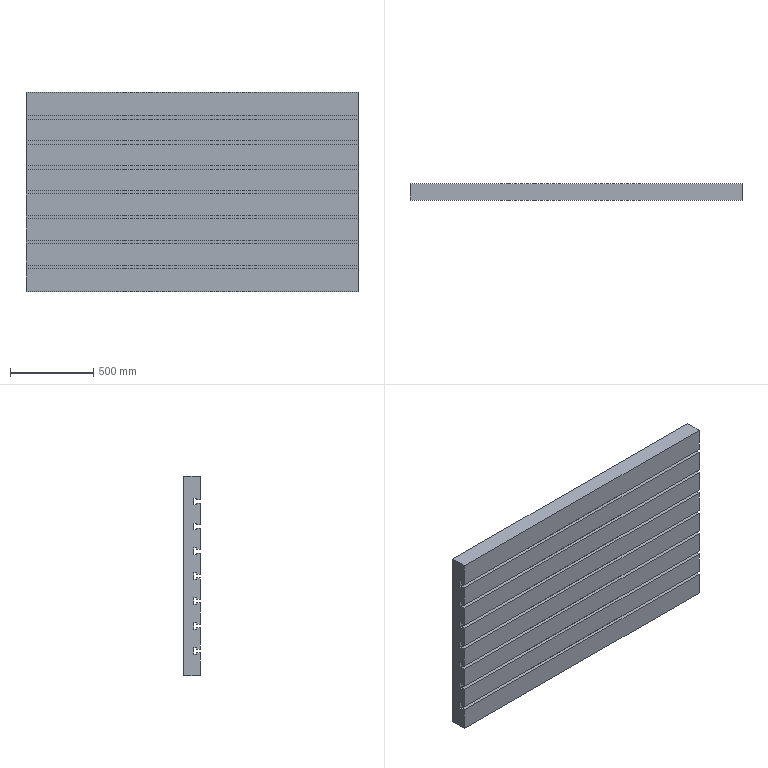CAM job | Mastercam | mm | 11 operations | part box 2000 x 100 x 1200
1. Contour (Ramp) | 10 - 10 平铣刀
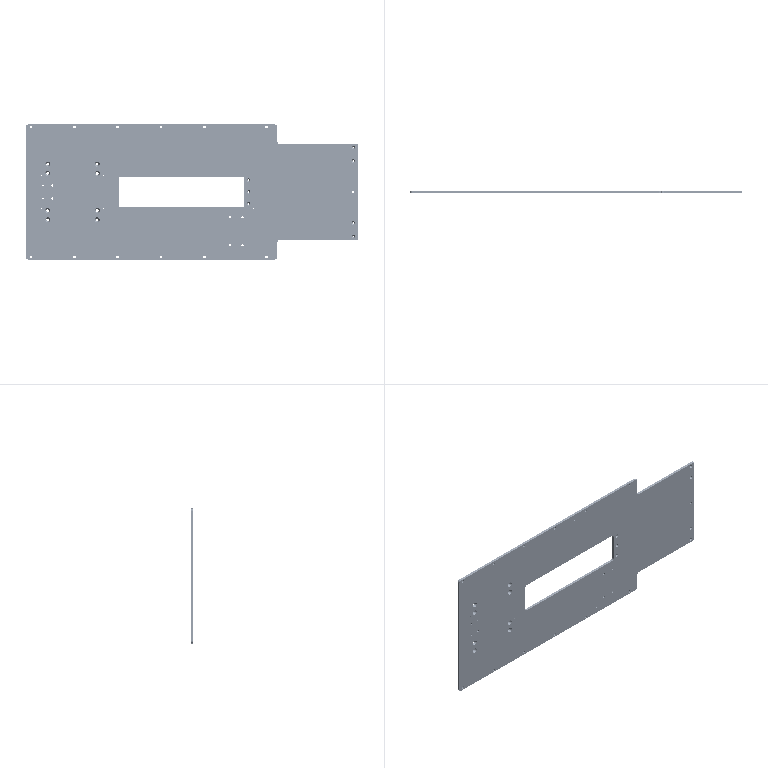2. Contour (Ramp) | 10 - 10 平铣刀
3. Contour (2D) | 10 - 10 平铣刀
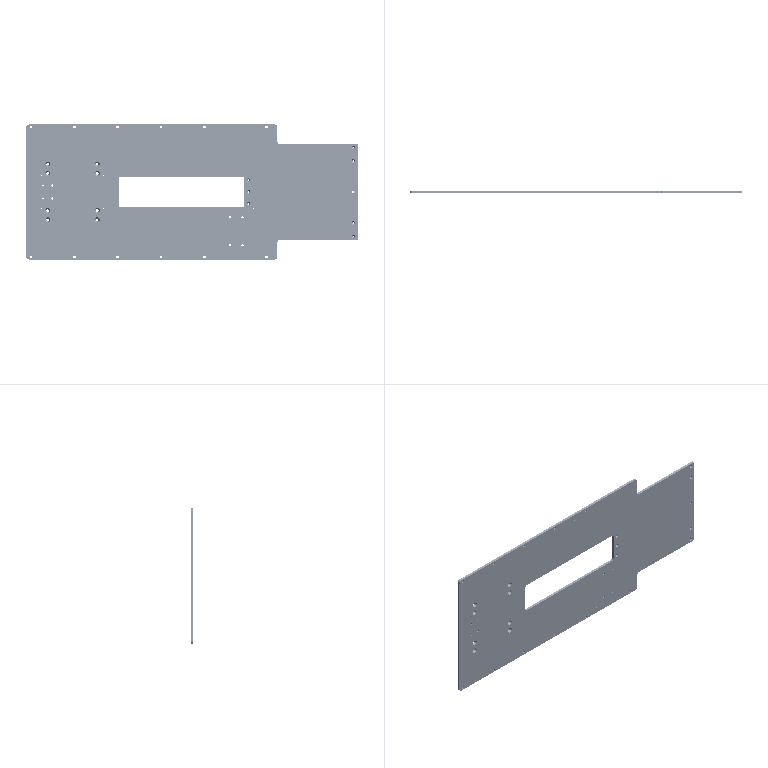4. Helix Bore | 6 - 6 平铣刀
5. 3D High Speed (Waterline) | 6 - 6 平铣刀
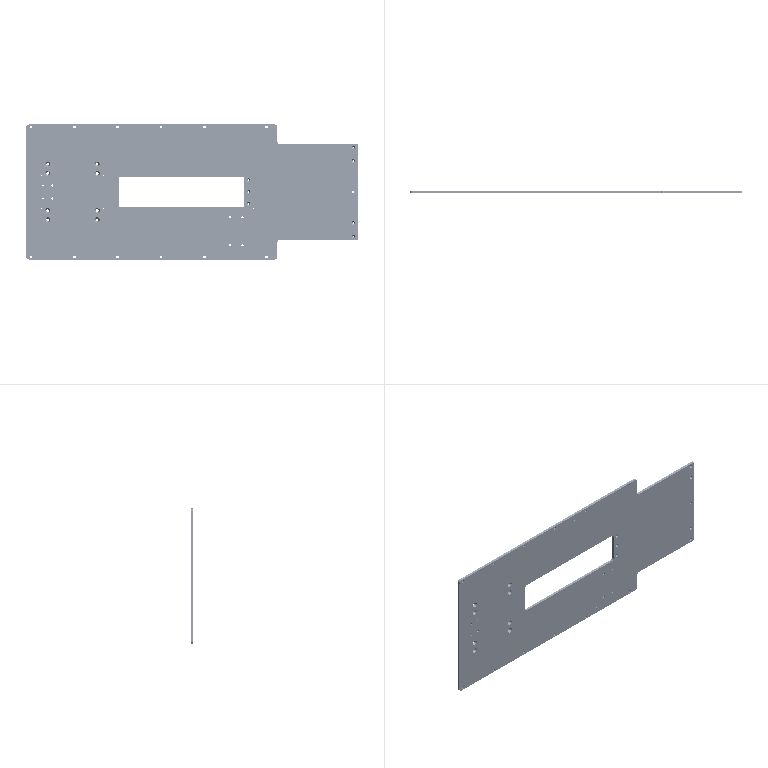6. Drill/Counterbore | 7 - 4 倒角刀
7. Contour (Ramp) | 10 - 10 平铣刀
8. Contour (2D) | 6 - 6 平铣刀
9. Drill/Counterbore | 7 - 4 倒角刀
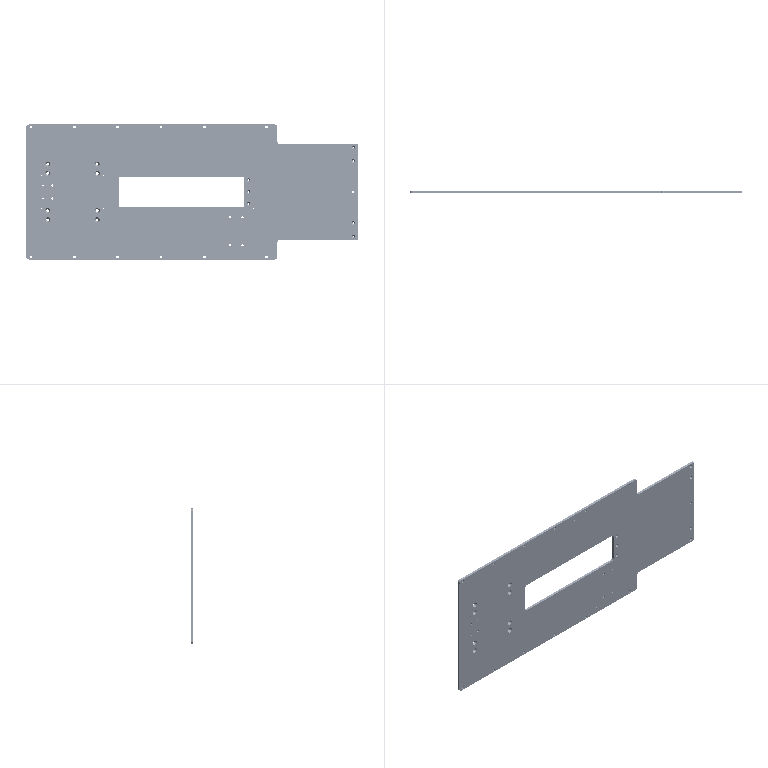10. Peck Drill | 1 - 5.5 钻头
11. 3D High Speed (Waterline) | 5 - 4 圆鼻铣刀